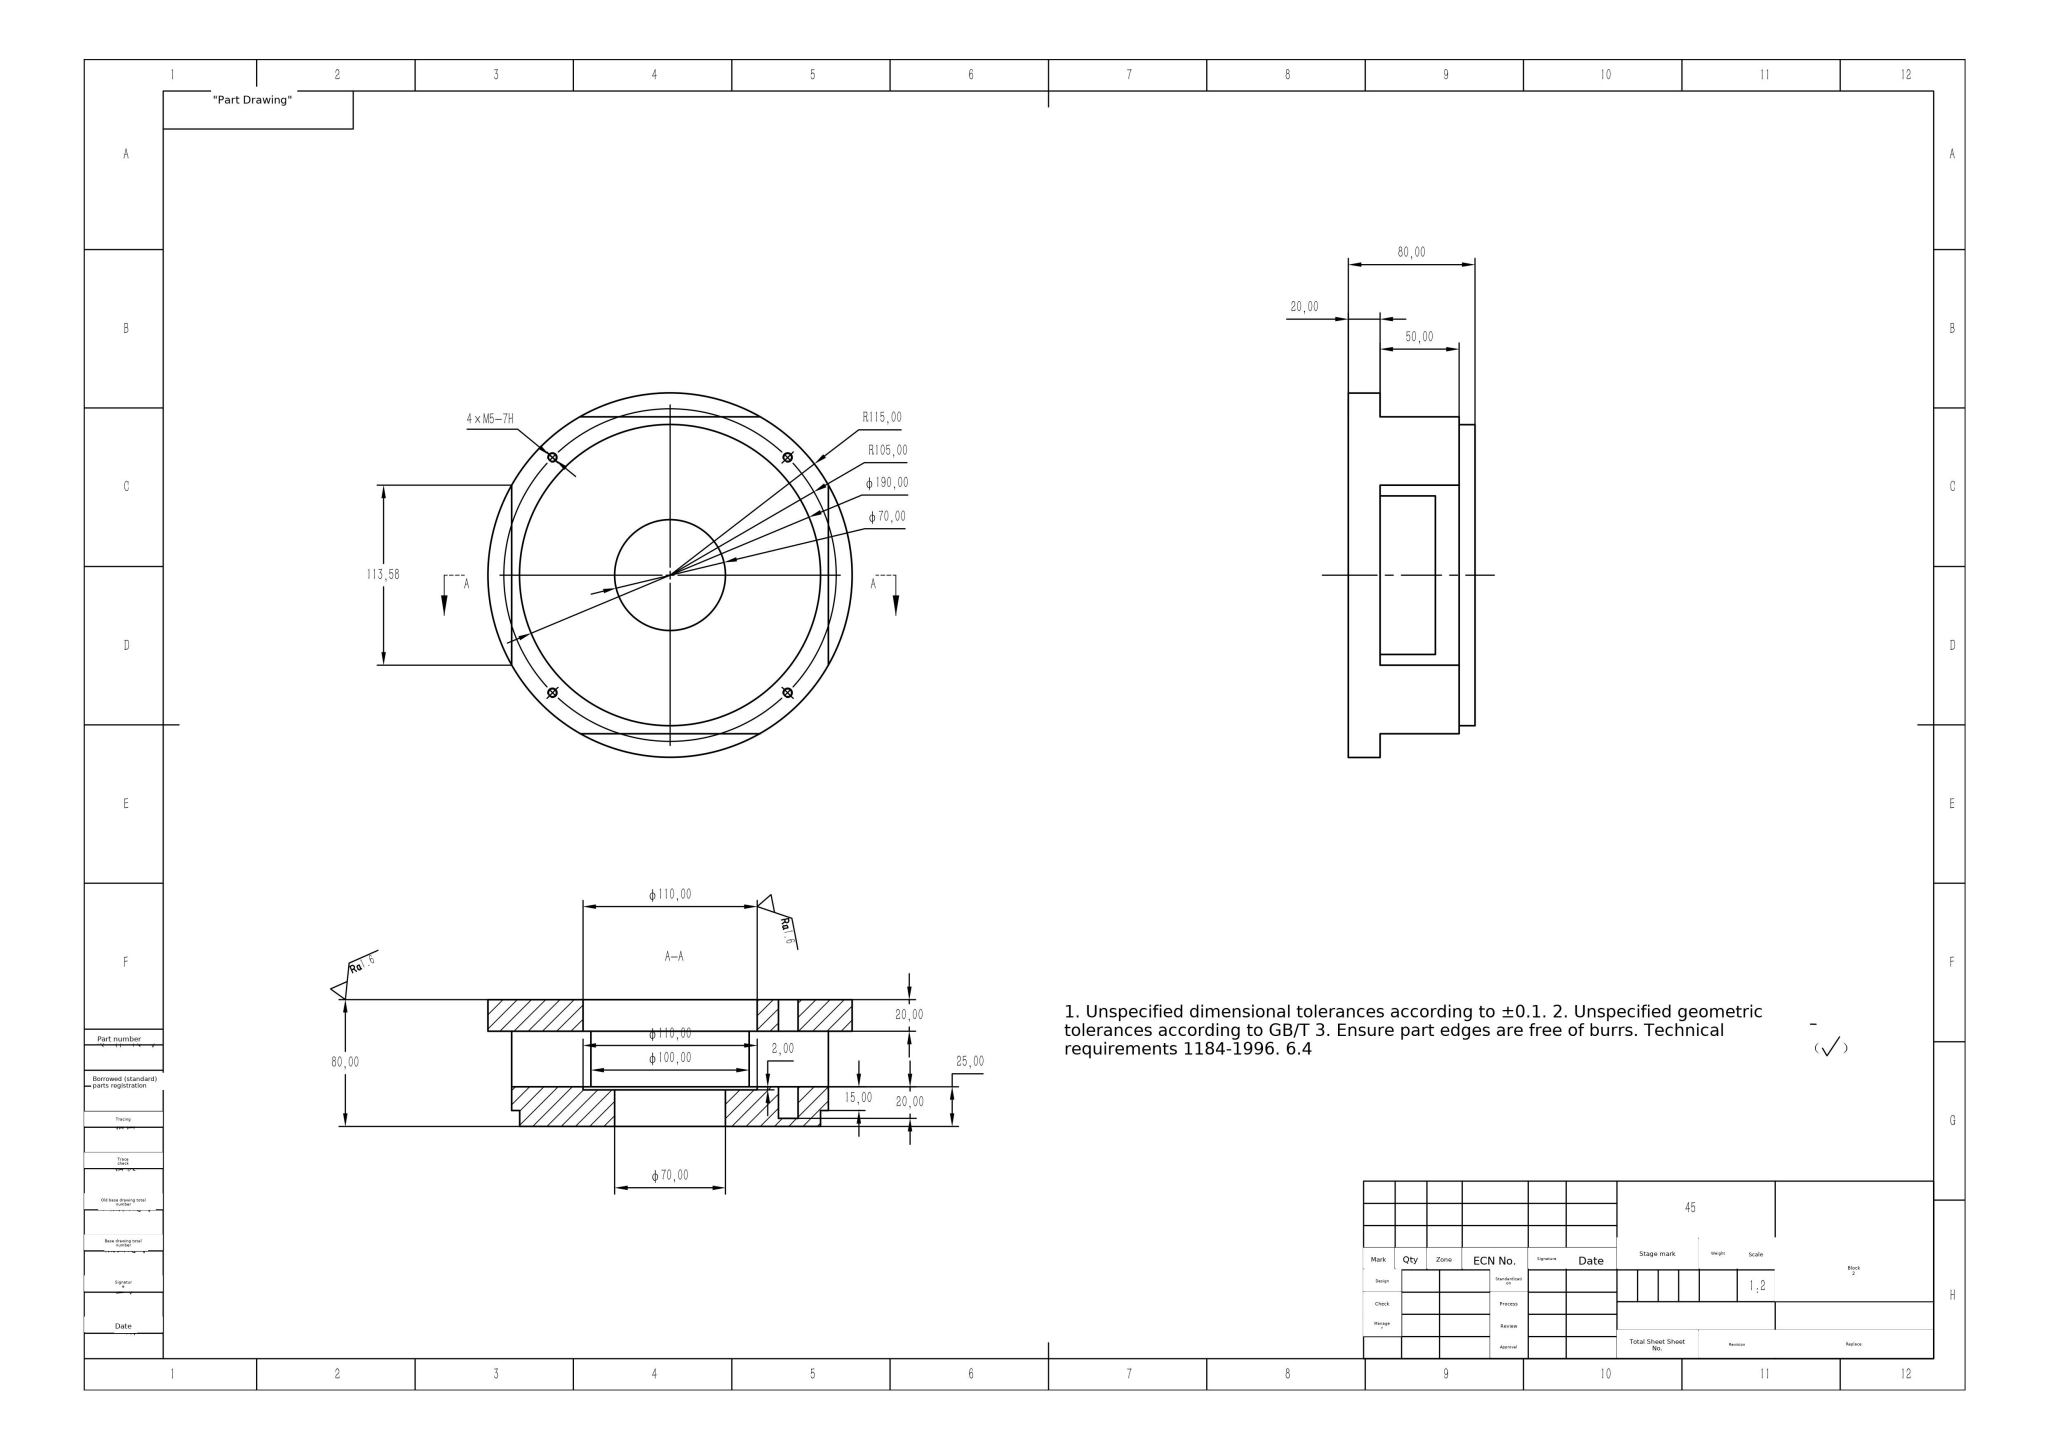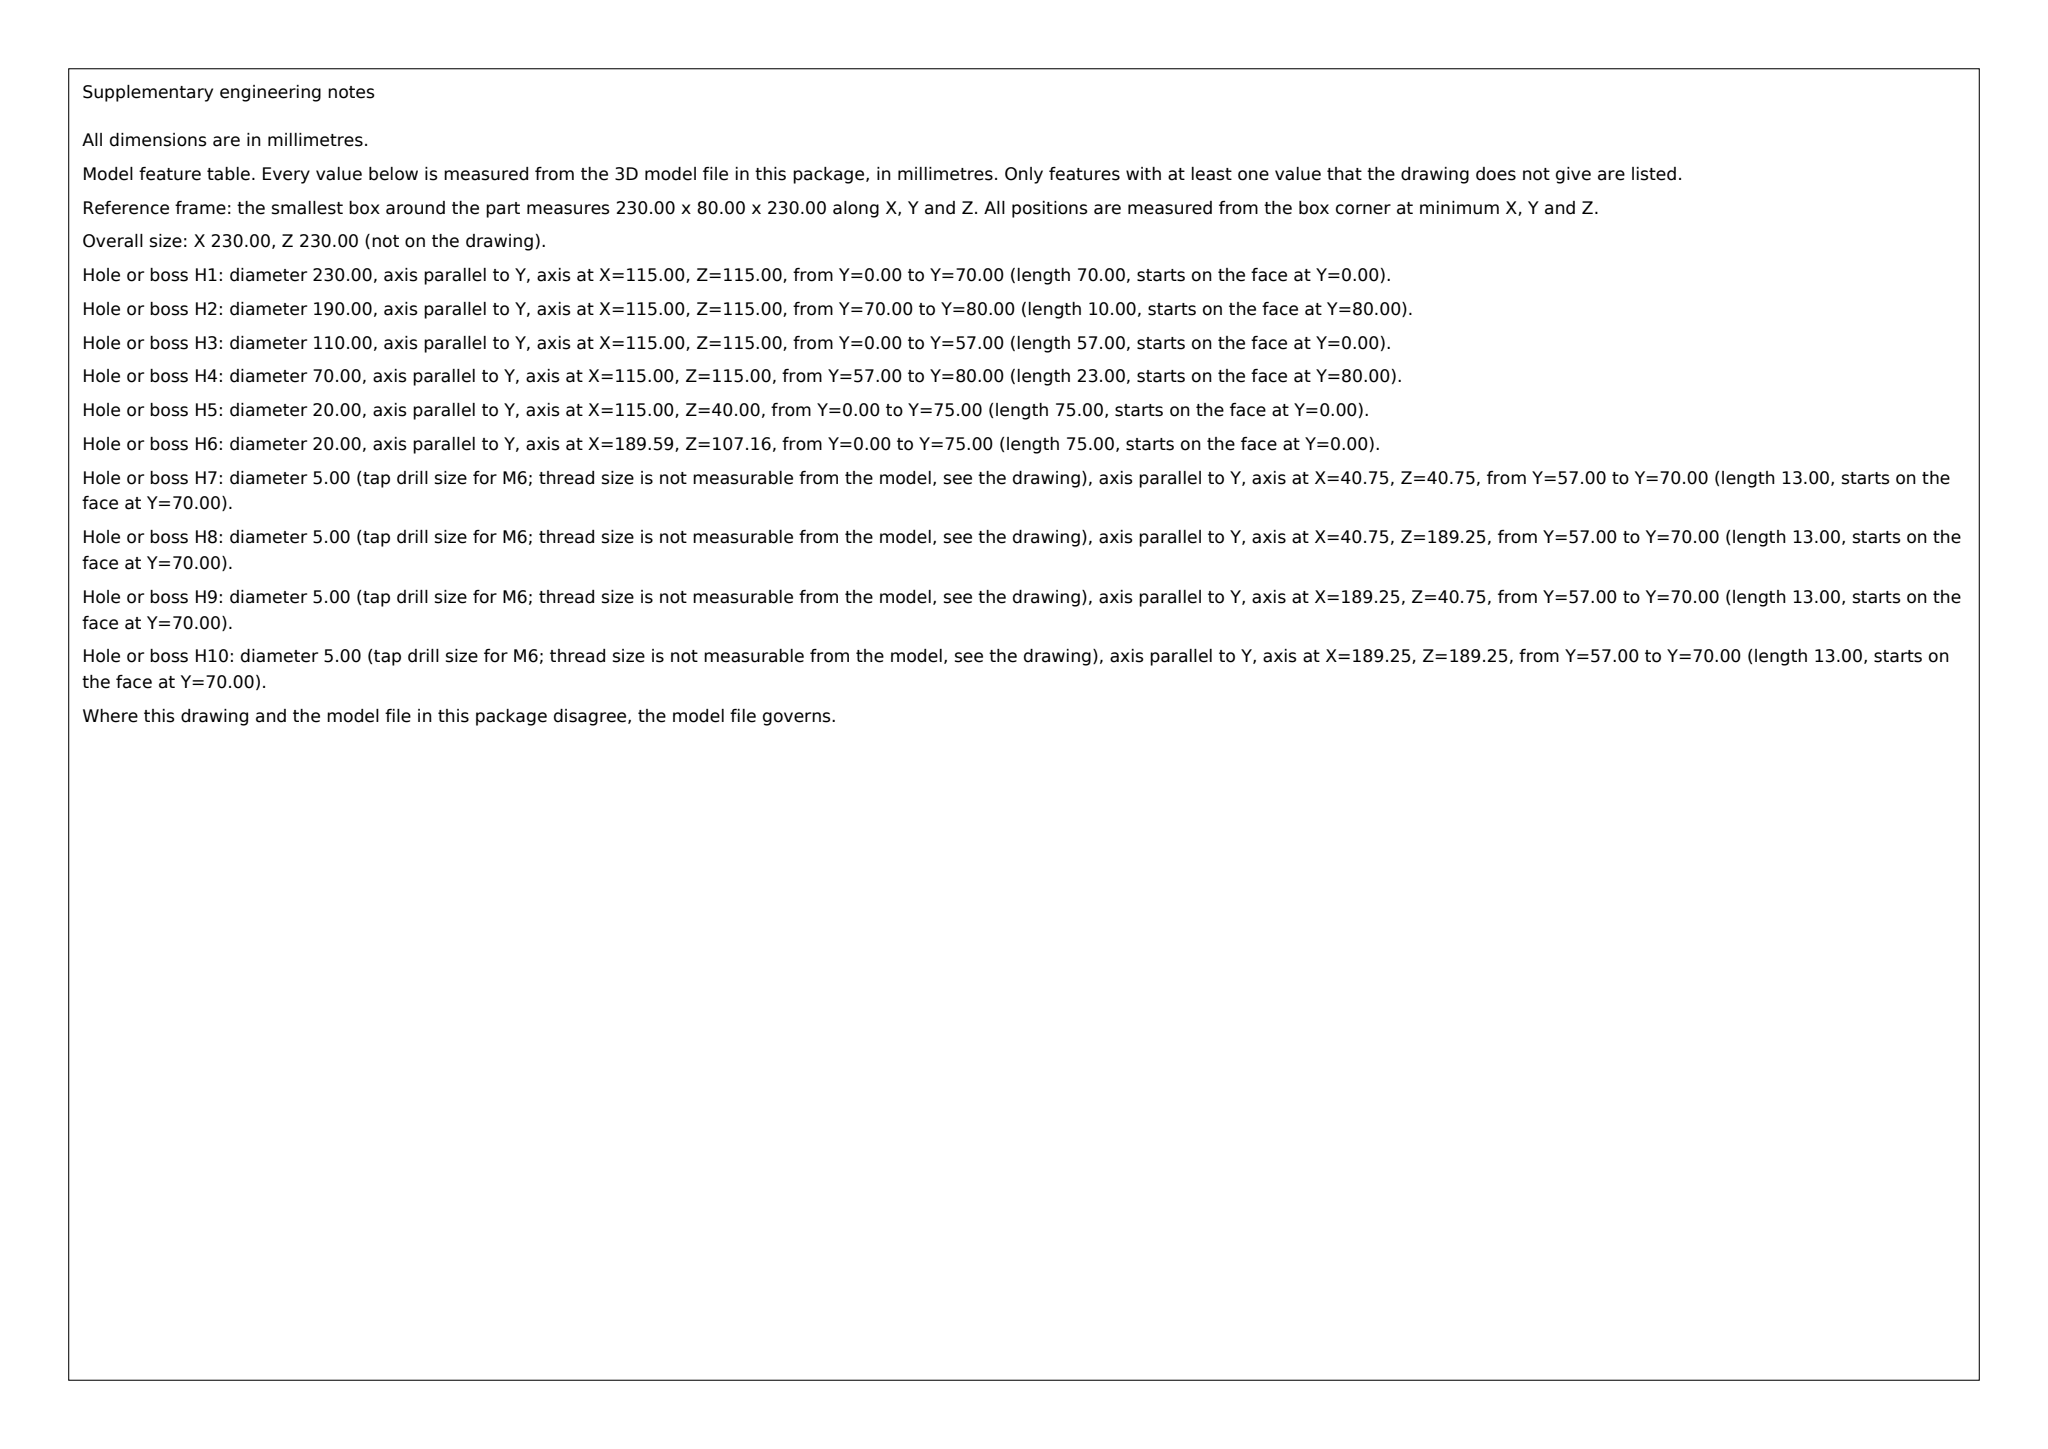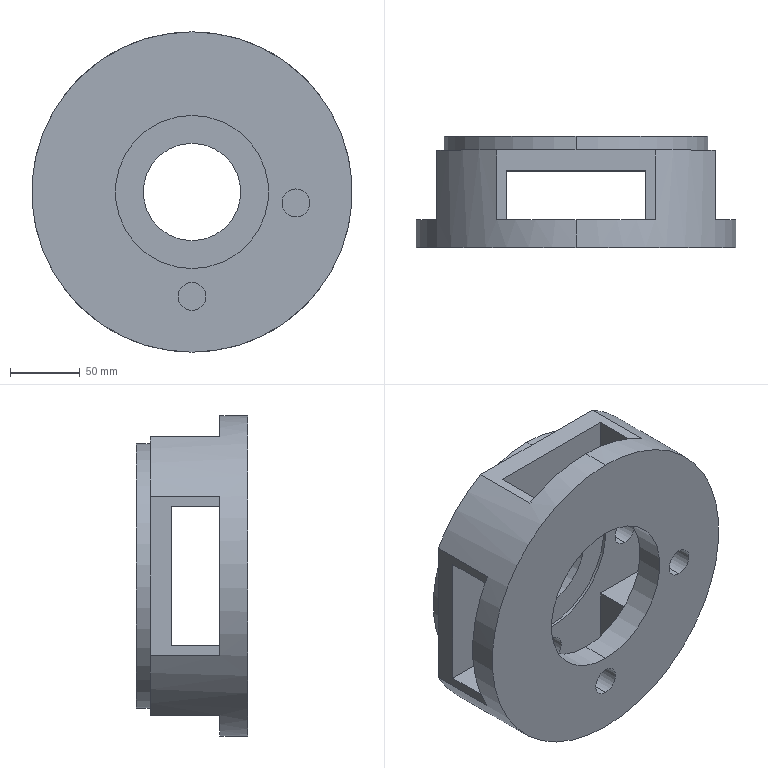Part | SolidWorks | mm | material 45 | 1 solid | 54 faces | box 230 x 80 x 230 mm | volume 1587783 mm3 | cylinder 26 | plane 20 | cone 8 | commonest cylinder face diameters 5 x8 20 x8 110 x4 190 x2 70 x2 230 x2